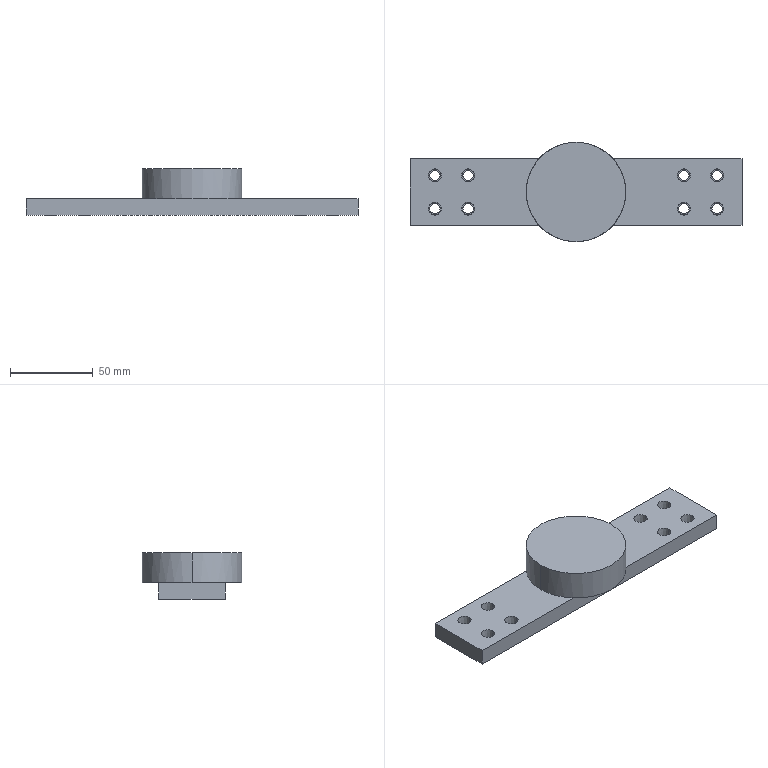Component | SolidWorks | Two-AxisRotation-1 | 1 solid | 52 faces | volume 127567 mm3 | cylinder 18 | plane 18 | cone 16 | commonest cylinder face diameters 6.147 x16 60 x2